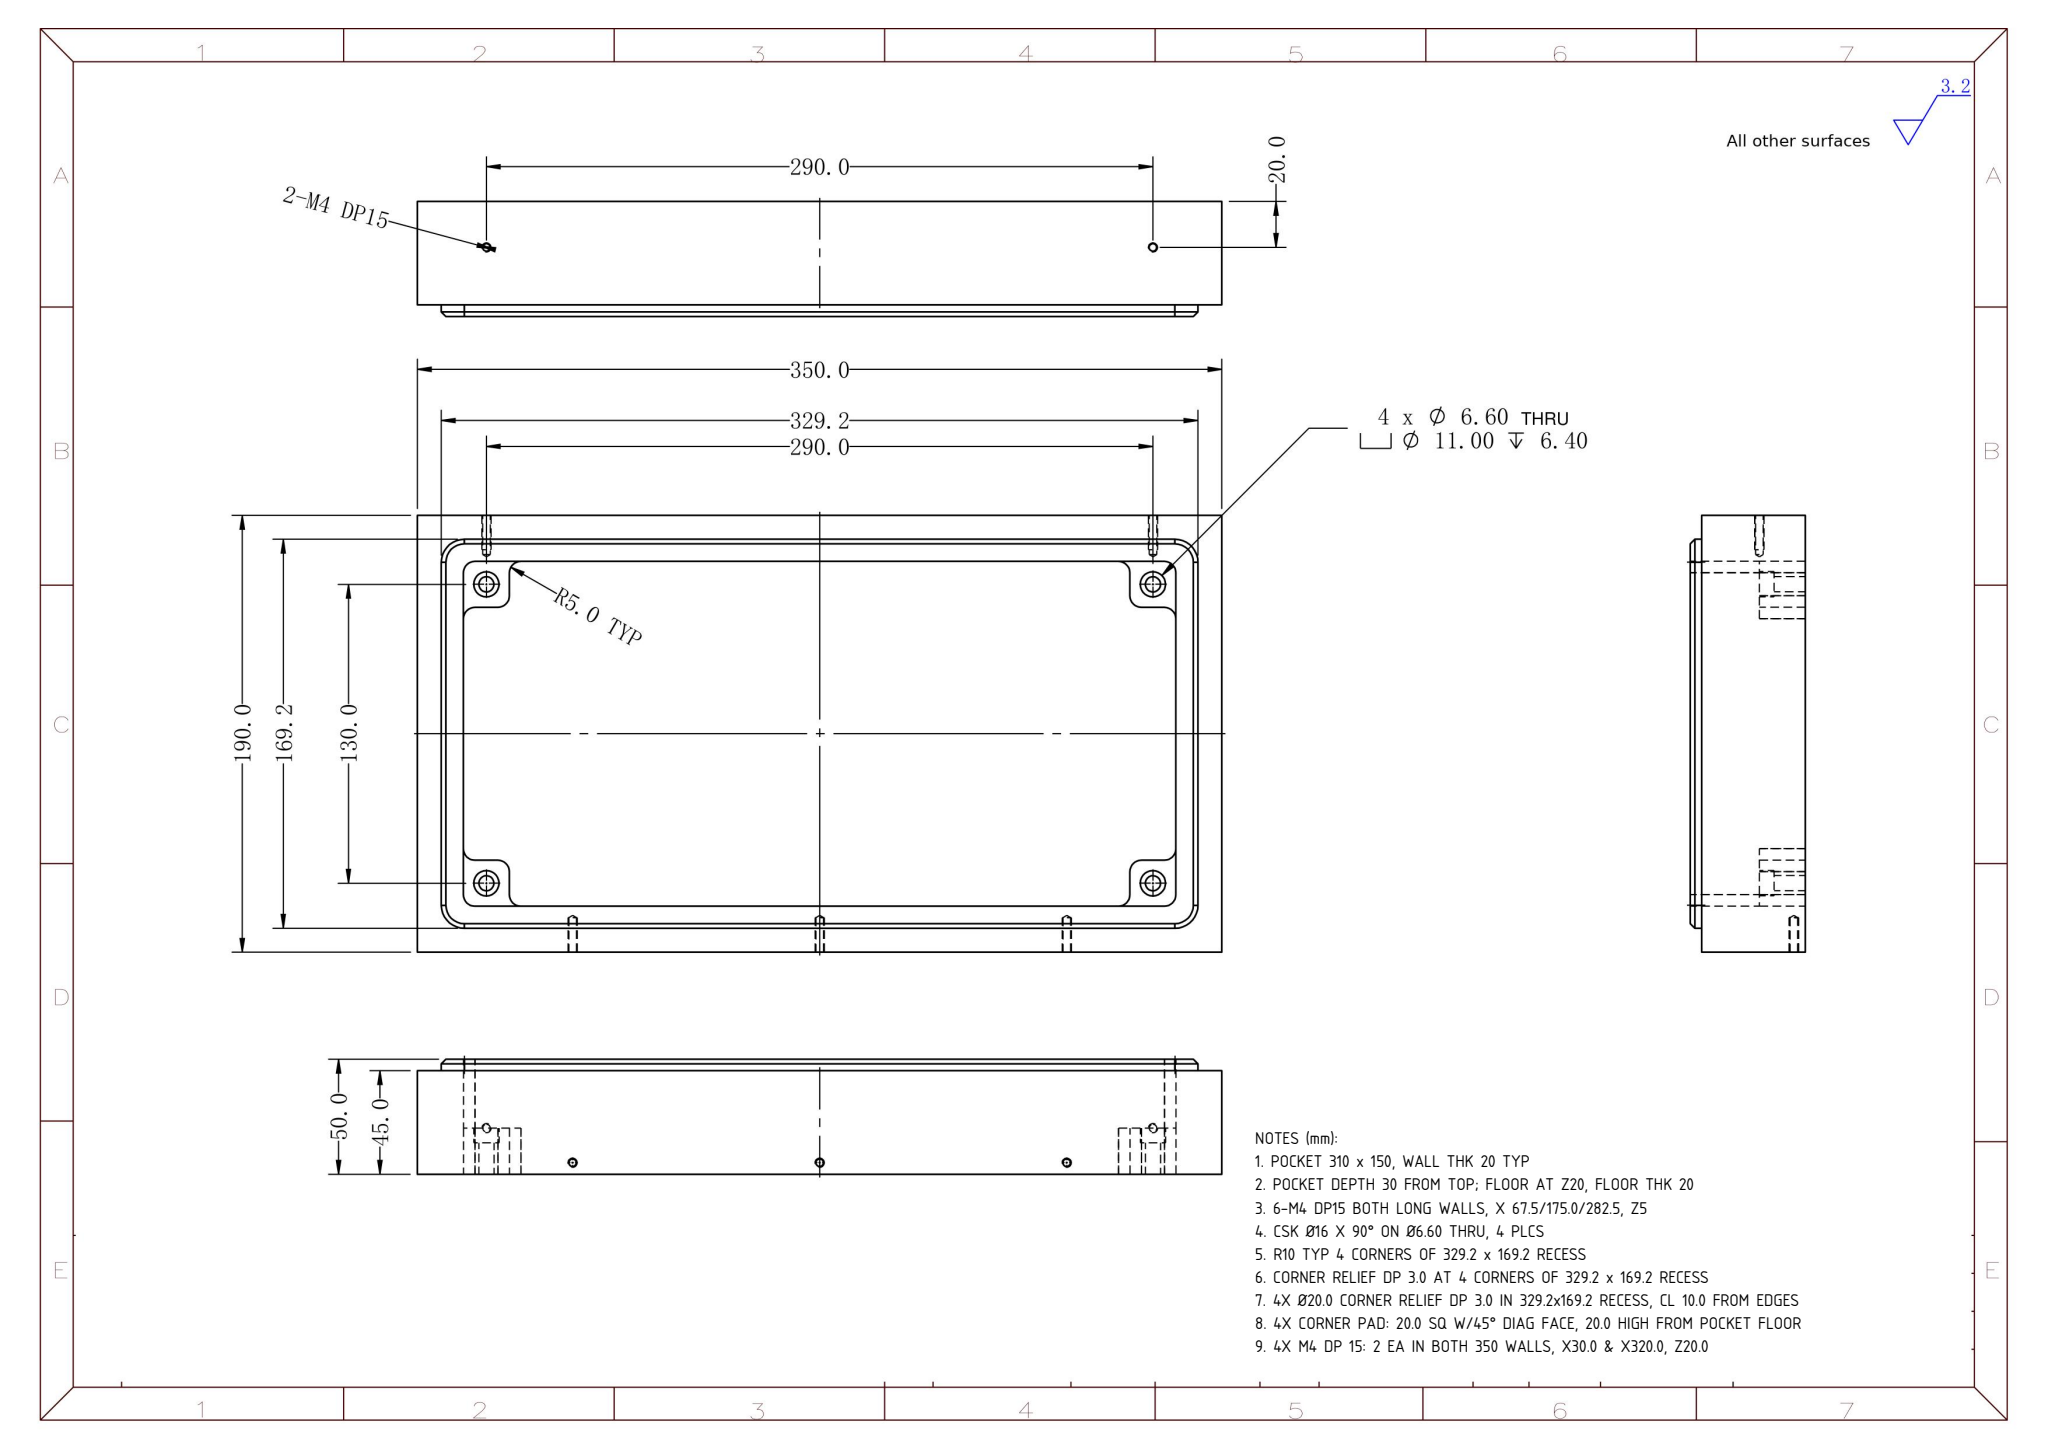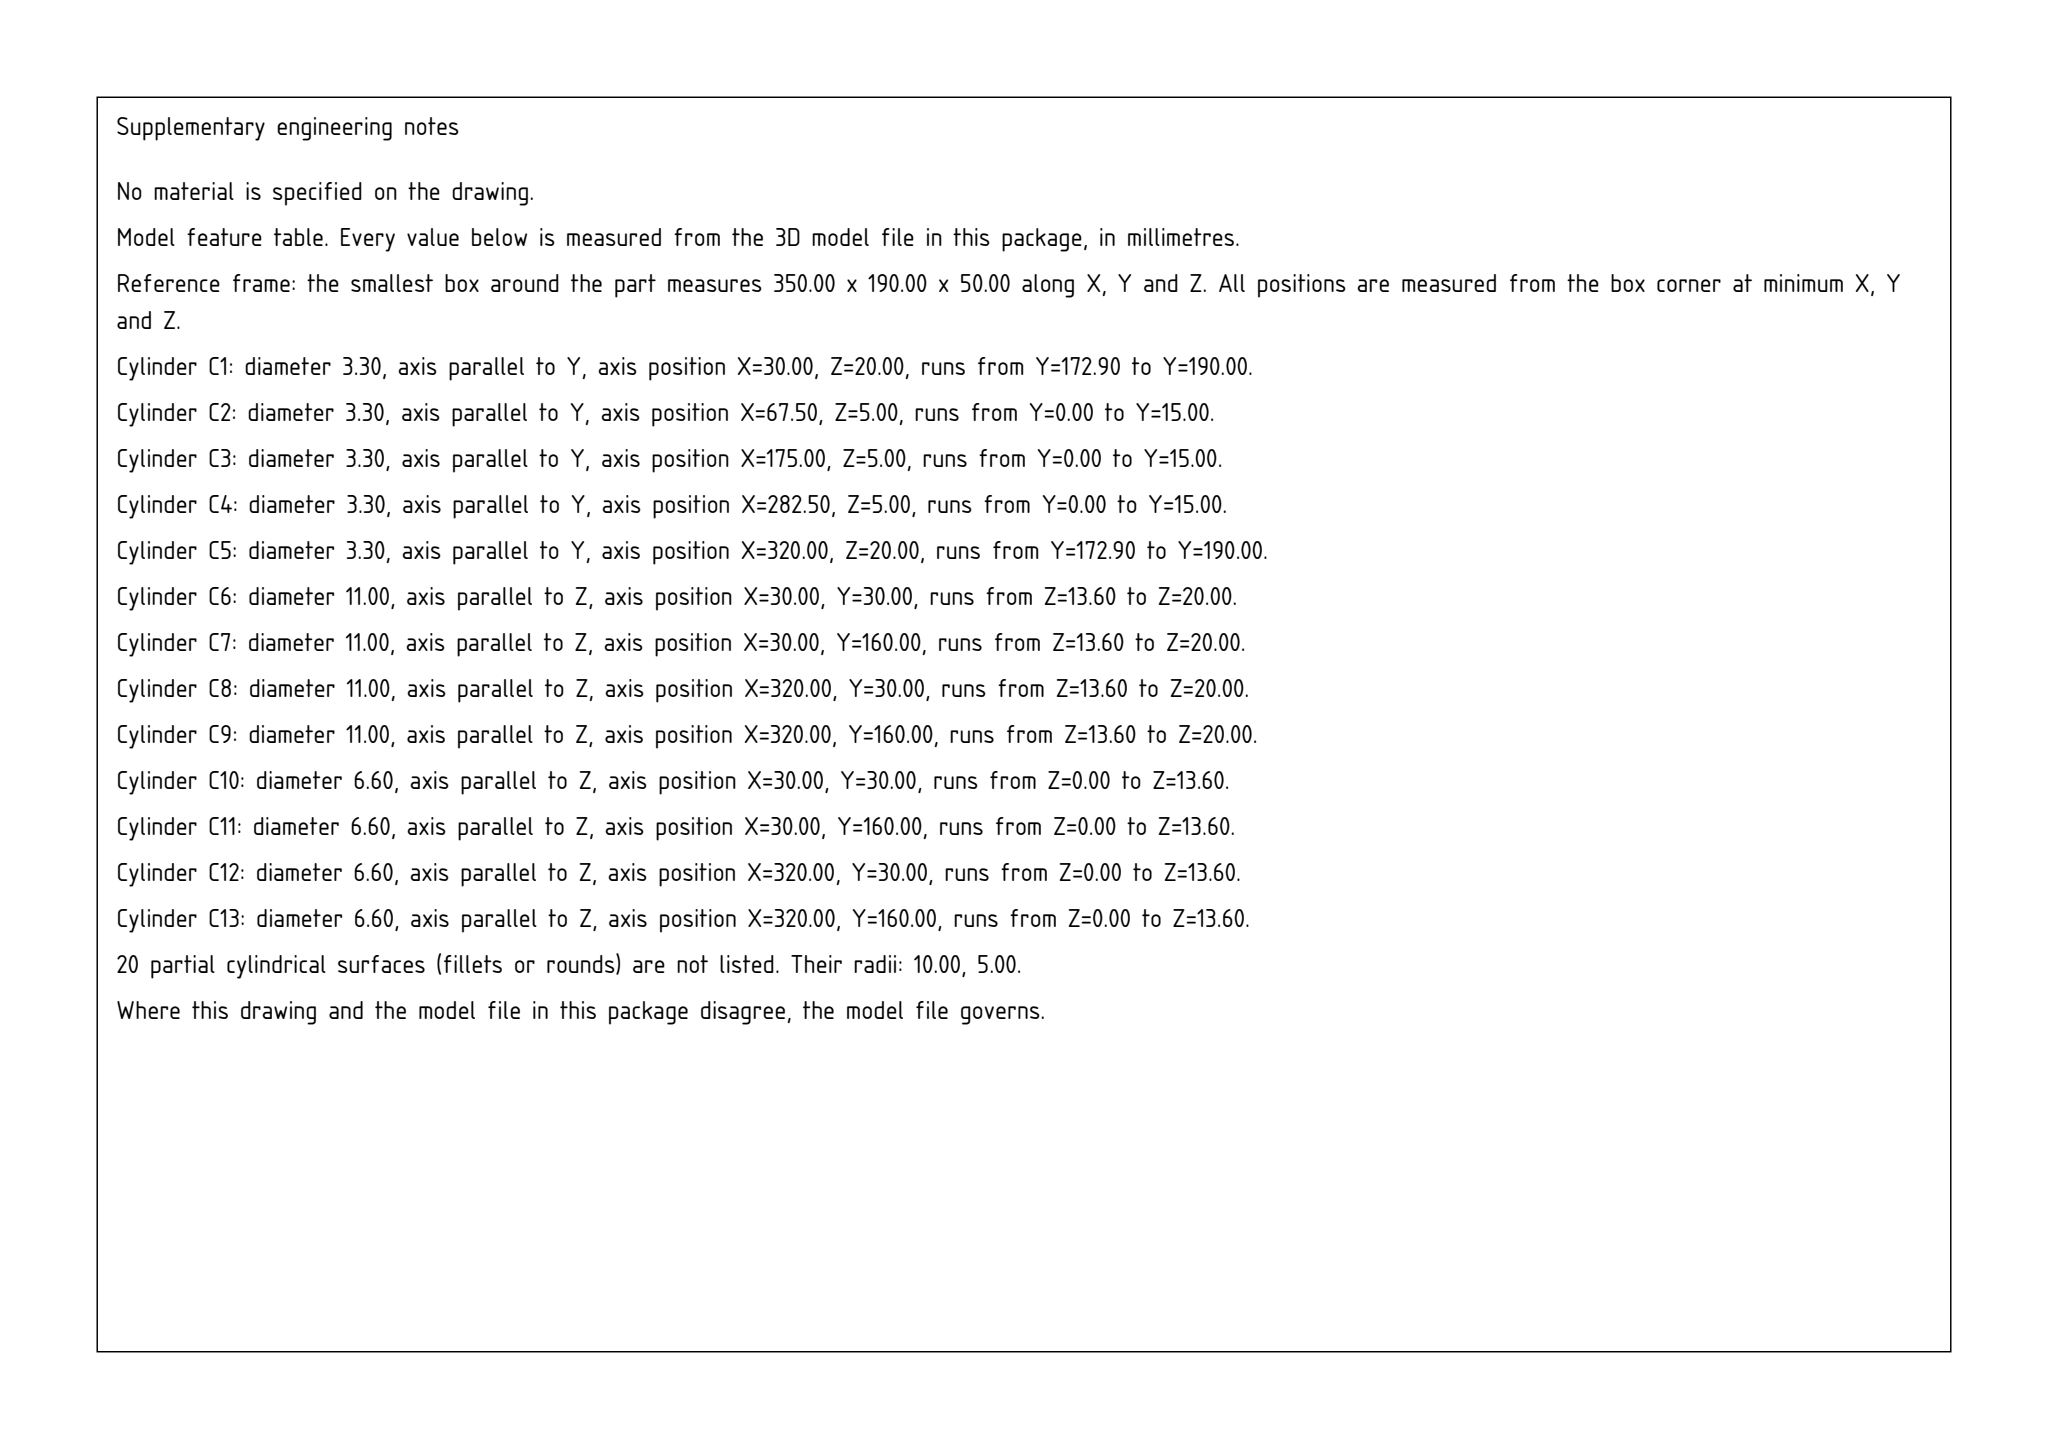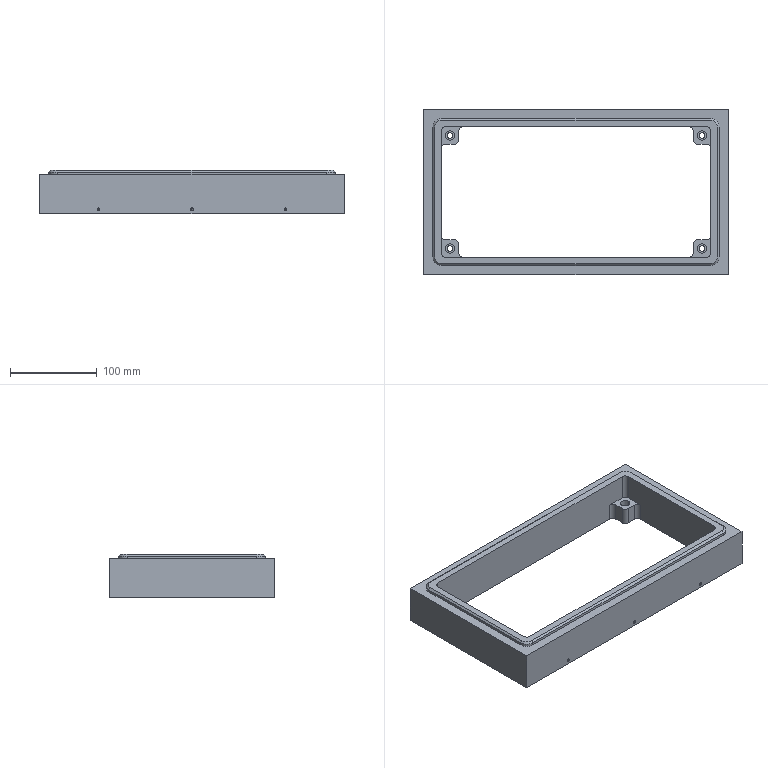Part | SolidWorks | mm | 1 solid | 95 faces | box 350 x 190 x 50 mm | volume 971711 mm3 | cylinder 46 | plane 35 | cone 14 | commonest cylinder face diameters 10 x16 3.3 x10 11 x8 6.6 x8 20 x4
Drawing notes:
POCKET 310 x 150, WALL THK 20 TYP | from the solid: x planes 20.0/330.0 and y planes 20.0/170.0 in 350x190 bbox
POCKET DEPTH 30 FROM TOP; FLOOR AT Z20, FLOOR THK 20 | from the solid: z plane 20.0 (pocket floor), bbox z=50
6-M4 DP15 BOTH LONG WALLS, X 67.5/175.0/282.5, Z5 | from the solid: Ø3.3 axis-y holes at x=67.5,175.0,282.5, z=5.0, len 15.0, 2 ea
CSK Ø16 X 90° ON Ø6.60 THRU, 4 PLCS | from the solid: cones 90° ref dia 16.0, qty 4, coaxial w/ Ø6.6 z-holes
R10 TYP 4 CORNERS OF 329.2 x 169.2 RECESS | from the solid: Ø20 z-cyl at (20.4,20.4),(20.4,169.6),(329.6,20.4),(329.6,169.6)
CORNER RELIEF DP 3.0 AT 4 CORNERS OF 329.2 x 169.2 RECESS | from the solid: Ø20 corner cylinders length 3.0 below top face z=50
4X Ø20.0 CORNER RELIEF DP 3.0 IN 329.2x169.2 RECESS, CL 10.0 FROM EDGES | from the solid: cyl dia 20.0 axis z len 3.0 at (20.4,20.4),(20.4,169.6),(329.6,20.4),(329.6,169.6); recess walls x=10.4/339.6, y=10.4/179.6
4X CORNER PAD: 20.0 SQ W/45° DIAG FACE, 20.0 HIGH FROM POCKET FLOOR | from the solid: planes x=40.0 & 310.0, y=40.0 & 150.0 vs pocket walls x=20/330, y=20/170; pad top plane z=20.0 (4), floor z=0; Ø6.6 len 13.6 + Ø11 cbore 6.4 = 20.0
4X M4 DP 15: 2 EA IN BOTH 350 WALLS, X30.0 & X320.0, Z20.0 | from the solid: cyl dia 3.3 axis y len 17.1 at (x30,z20) count 2 and (x320,z20) count 2 = 4 total, one pair per long wall
build123d program:
from build123d import *

# Parameters (mm, degrees)
SKETCH1_W                                       = 350
SKETCH1_H                                       = 190
BOSS_EXTRUDE1_DEPTH                             = 25
SKETCH2_W                                       = 310
SKETCH2_H                                       = 150
CUT_EXTRUDE1_DEPTH                              = 206.305
SKETCH3_W                                       = 20
SKETCH3_H                                       = 20
BOSS_EXTRUDE2_DEPTH                             = 50
SKETCH6_W                                       = 350
SKETCH6_H                                       = 190
CUT_EXTRUDE2_DEPTH                              = 5
SKETCH7_W                                       = 20
SKETCH7_H                                       = 20
CUT_EXTRUDE3_DEPTH                              = 30
M6_HEX_SOCKET_HEAD_CAP_SCREW_CBORE2_D           = 6.6
M6_HEX_SOCKET_HEAD_CAP_SCREW_CBORE2_CBORE_D     = 11
M6_HEX_SOCKET_HEAD_CAP_SCREW_CBORE2_CBORE_DEPTH = 6.4
FILLET2_R                                       = 5
CHAMFER1_SIZE                                   = 2
M4_TAPPED_HOLE1_D                               = 3.3
M4_TAPPED_HOLE1_DEPTH                           = 15
M4_TAPPED_HOLE1_TIP                             = 0.9914
M4_TAPPED_HOLE2_D                               = 3.3
M4_TAPPED_HOLE2_DEPTH                           = 17.1
M4_TAPPED_HOLE2_TIP                             = 0.9914


with BuildPart() as part:
    # Sketch1 → Boss-Extrude1 (new, symmetric)
    with BuildSketch(Plane.XY):
        Rectangle(SKETCH1_W, SKETCH1_H)
    extrude(amount=BOSS_EXTRUDE1_DEPTH, both=True)

    # Sketch2 → Cut-Extrude1 (cut, through all)
    with BuildSketch(Plane.XY.offset(25)):
        Rectangle(SKETCH2_W, SKETCH2_H)
    extrude(amount=-CUT_EXTRUDE1_DEPTH, mode=Mode.SUBTRACT)

    # Sketch3 → Boss-Extrude2 (add)
    with BuildSketch(Plane.XY.offset(25)):
        with Locations((145, 65)):
            Rectangle(SKETCH3_W, SKETCH3_H)
        with Locations((145, -65)):
            Rectangle(SKETCH3_W, SKETCH3_H)
        with Locations((-145, -65)):
            Rectangle(SKETCH3_W, SKETCH3_H)
        with Locations((-145, 65)):
            Rectangle(SKETCH3_W, SKETCH3_H)
    extrude(amount=-BOSS_EXTRUDE2_DEPTH)

    # Sketch6 → Cut-Extrude2 (cut)
    with BuildSketch(Plane.XY.offset(25)):
        Rectangle(SKETCH6_W, SKETCH6_H)
        with BuildLine():
            Line((154.6, -84.6), (-154.6, -84.6))
            ThreePointArc((-154.6, -84.6), (-161.671, -81.671), (-164.6, -74.6))
            Line((-164.6, -74.6), (-164.6, 74.6))
            ThreePointArc((-164.6, 74.6), (-161.671, 81.671), (-154.6, 84.6))
            Line((-154.6, 84.6), (154.6, 84.6))
            ThreePointArc((154.6, 84.6), (161.671, 81.671), (164.6, 74.6))
            Line((164.6, 74.6), (164.6, -74.6))
            ThreePointArc((164.6, -74.6), (161.671, -81.671), (154.6, -84.6))
        make_face(mode=Mode.SUBTRACT)
    extrude(amount=-CUT_EXTRUDE2_DEPTH, mode=Mode.SUBTRACT)

    # Sketch7 → Cut-Extrude3 (cut)
    with BuildSketch(Plane.XY.offset(25)):
        with Locations((-145, 65)):
            Rectangle(SKETCH7_W, SKETCH7_H)
        with Locations((145, 65)):
            Rectangle(SKETCH7_W, SKETCH7_H)
        with Locations((145, -65)):
            Rectangle(SKETCH7_W, SKETCH7_H)
        with Locations((-145, -65)):
            Rectangle(SKETCH7_W, SKETCH7_H)
    extrude(amount=-CUT_EXTRUDE3_DEPTH, mode=Mode.SUBTRACT)

    # M6 Hex Socket Head Cap Screw CBORE2 (through all)
    with Locations(Plane.XY.offset(-5)):
        with Locations((-145, 65), (145, 65), (-145, -65), (145, -65)):
            CounterBoreHole(M6_HEX_SOCKET_HEAD_CAP_SCREW_CBORE2_D / 2, M6_HEX_SOCKET_HEAD_CAP_SCREW_CBORE2_CBORE_D / 2, M6_HEX_SOCKET_HEAD_CAP_SCREW_CBORE2_CBORE_DEPTH)

    # Fillet2
    fillet2_edges = [part.edges().sort_by_distance(p)[0] for p in [
        (-155, 75, 10),
        (155, 75, 10),
        (155, -75, 10),
        (-155, -75, 10),
        (155, 55, -15),
        (135, 55, -15),
        (135, 75, -15),
        (155, -55, -15),
        (135, -75, -15),
        (135, -55, -15),
        (-135, -75, -15),
        (-155, -55, -15),
        (-135, -55, -15),
        (-135, 75, -15),
        (-135, 55, -15),
        (-155, 55, -15),
    ]]
    fillet(fillet2_edges, radius=FILLET2_R)

    # Chamfer1
    chamfer1_edges = [part.edges().sort_by_distance(p)[0] for p in [
        (-161.671, -81.671, 25),
        (-164.6, 0, 25),
        (-161.671, 81.671, 25),
        (0, 84.6, 25),
        (161.671, 81.671, 25),
        (164.6, 0, 25),
        (161.671, -81.671, 25),
        (0, -84.6, 25),
    ]]
    chamfer(chamfer1_edges, length=CHAMFER1_SIZE)

    # M4 Tapped Hole1
    with Locations(Plane(origin=(0, -95, 0), x_dir=(-1, 0, 0), z_dir=(0, -1, 0))):
        with Locations((107.5, 20), (0, 20), (-107.5, 20)):
            Hole(M4_TAPPED_HOLE1_D / 2, depth=M4_TAPPED_HOLE1_DEPTH)
            with Locations((0, 0, -(M4_TAPPED_HOLE1_DEPTH + M4_TAPPED_HOLE1_TIP / 2))):  # 118° drill point
                Cone(0, M4_TAPPED_HOLE1_D / 2, M4_TAPPED_HOLE1_TIP, mode=Mode.SUBTRACT)

    # M4 Tapped Hole2
    with Locations(Plane(origin=(0, 95, 0), x_dir=(1, 0, 0), z_dir=(0, 1, 0))):
        with Locations((-145, 5), (145, 5)):
            Hole(M4_TAPPED_HOLE2_D / 2, depth=M4_TAPPED_HOLE2_DEPTH)
            with Locations((0, 0, -(M4_TAPPED_HOLE2_DEPTH + M4_TAPPED_HOLE2_TIP / 2))):  # 118° drill point
                Cone(0, M4_TAPPED_HOLE2_D / 2, M4_TAPPED_HOLE2_TIP, mode=Mode.SUBTRACT)


solid = part.part